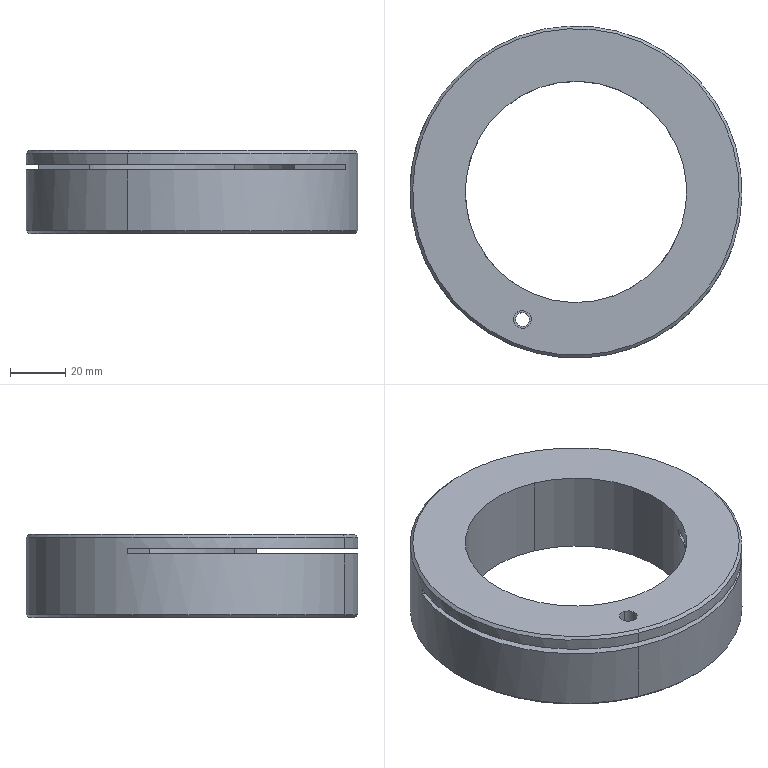Component | SolidWorks | 8TC-A17001-20-07LockingSleeve-1 | 1 solid | 34 faces | box 120 x 120 x 30 mm | volume 180598 mm3 | cylinder 16 | cone 12 | plane 6 | commonest cylinder face diameters 3.3 x8 5 x2 6.4 x2 80 x2 120 x2 | material #45
build123d program:
from build123d import *

# Parameters (mm, degrees)
SKETCH1_R                      = 60
SKETCH1_R_2                    = 40
BOSS_EXTRUDE1_DEPTH            = 15
SKETCH2_W                      = 60
SKETCH2_H                      = 2
CUT_EXTRUDE1_DEPTH             = 60
F_6_4_6_4_DIAMETER_HOLE1_D     = 6.4
F_6_4_6_4_DIAMETER_HOLE1_DEPTH = 5
M6_TAPPED_HOLE1_D              = 5
CHAMFER1_SIZE                  = 1
M4_TAPPED_HOLE1_D              = 3.3
M4_TAPPED_HOLE1_DEPTH          = 18
M4_TAPPED_HOLE1_TIP            = 0.9914


with BuildPart() as part:
    # Sketch1 → Boss-Extrude1 (new, symmetric)
    with BuildSketch(Plane(origin=(0, 0, 0), x_dir=(1, 0, 0), z_dir=(0, 1, 0))):
        with Locations(Location((0, 0, 0), (0, 0, 270))):
            Circle(SKETCH1_R)
        with Locations(Location((0, 0, 0), (0, 0, 270))):
            Circle(SKETCH1_R_2, mode=Mode.SUBTRACT)
    extrude(amount=BOSS_EXTRUDE1_DEPTH, both=True)

    # Sketch2 → Cut-Extrude1 (cut, symmetric)
    with BuildSketch(Plane(origin=(0, 0, 0), x_dir=(0, 0, -1), z_dir=(1, 0, 0))):
        with Locations((-30, 9)):
            Rectangle(SKETCH2_W, SKETCH2_H)
    extrude(amount=CUT_EXTRUDE1_DEPTH, both=True, mode=Mode.SUBTRACT)

    # 6.4 _6.4_ Diameter Hole1
    with Locations(Plane(origin=(0, 15, 0), x_dir=(1, 0, 0), z_dir=(0, 1, 0))):
        with Locations((0, -50)):
            Hole(F_6_4_6_4_DIAMETER_HOLE1_D / 2, depth=F_6_4_6_4_DIAMETER_HOLE1_DEPTH)

    # M6 Tapped Hole1 (through all)
    with Locations(Plane(origin=(0, 8, 0), x_dir=(1, 0, 0), z_dir=(0, 1, 0))):
        with Locations((0, -50)):
            Hole(M6_TAPPED_HOLE1_D / 2)

    # Chamfer1
    chamfer1_edges = [part.edges().sort_by_distance(p)[0] for p in [
        (0, -15, -60),
        (0, 15, -60),
    ]]
    chamfer(chamfer1_edges, length=CHAMFER1_SIZE)

    # M4 Tapped Hole1
    with Locations(Plane(origin=(0, -15, 0), x_dir=(-1, 0, 0), z_dir=(0, -1, 0))):
        with Locations((-35.355, 35.355), (35.355, 35.355), (35.355, -35.355), (-35.355, -35.355)):
            Hole(M4_TAPPED_HOLE1_D / 2, depth=M4_TAPPED_HOLE1_DEPTH)
            with Locations((0, 0, -(M4_TAPPED_HOLE1_DEPTH + M4_TAPPED_HOLE1_TIP / 2))):  # 118° drill point
                Cone(0, M4_TAPPED_HOLE1_D / 2, M4_TAPPED_HOLE1_TIP, mode=Mode.SUBTRACT)


solid = part.part

# Placed as in the assembly
solid = solid.moved(Location((733.029, 200.722, 253.5), (90, -22.788, 0)))
STEP:
#1=COLOUR_RGB('',0.7922,0.8196,0.9333);
#2=FILL_AREA_STYLE_COLOUR('',#1);
#3=FILL_AREA_STYLE('',(#2));
#4=SURFACE_STYLE_FILL_AREA(#3);
#5=SURFACE_SIDE_STYLE('',(#4));
#6=SURFACE_STYLE_USAGE(.BOTH.,#5);
#7=PRESENTATION_STYLE_ASSIGNMENT((#6));
#8=CARTESIAN_POINT('',(30.657,8.587,10.098));
#9=VERTEX_POINT('',#8);
#10=CARTESIAN_POINT('',(30.707,8.706,10.098));
#11=VERTEX_POINT('',#10);
#12=CARTESIAN_POINT('',(30.682,8.647,10.098));
#13=DIRECTION('',(-0.,-0.,-1.));
#14=DIRECTION('',(0.3873,0.9219,0.));
#15=AXIS2_PLACEMENT_3D('',#12,#13,#14);
#16=CIRCLE('',#15,0.06496);
#17=EDGE_CURVE('',#9,#11,#16,.T.);
#18=ORIENTED_EDGE('',*,*,#17,.F.);
#19=CARTESIAN_POINT('',(30.657,8.587,9.39));
#20=VERTEX_POINT('',#19);
#21=CARTESIAN_POINT('',(30.657,8.587,9.39));
#22=DIRECTION('',(-0.,-0.,-1.));
#23=VECTOR('',#22,39.37);
#24=LINE('',#21,#23);
#25=EDGE_CURVE('',#9,#20,#24,.T.);
#26=ORIENTED_EDGE('',*,*,#25,.T.);
#27=CARTESIAN_POINT('',(30.707,8.706,9.39));
#28=VERTEX_POINT('',#27);
#29=CARTESIAN_POINT('',(30.682,8.647,9.39));
#30=DIRECTION('',(-0.,-0.,-1.));
#31=DIRECTION('',(0.3873,0.9219,0.));
#32=AXIS2_PLACEMENT_3D('',#29,#30,#31);
#33=CIRCLE('',#32,0.06496);
#34=EDGE_CURVE('',#20,#28,#33,.T.);
#35=ORIENTED_EDGE('',*,*,#34,.T.);
#36=CARTESIAN_POINT('',(30.707,8.706,9.39));
#37=DIRECTION('',(-0.,-0.,-1.));
#38=VECTOR('',#37,39.37);
#39=LINE('',#36,#38);
#40=EDGE_CURVE('',#11,#28,#39,.T.);
#41=ORIENTED_EDGE('',*,*,#40,.F.);
#42=EDGE_LOOP('',(#18,#26,#35,#41));
#43=FACE_OUTER_BOUND('',#42,.T.);
#44=CARTESIAN_POINT('',(30.682,8.647,9.39));
#45=DIRECTION('',(-0.,-0.,-1.));
#46=DIRECTION('',(0.3873,0.9219,0.));
#47=AXIS2_PLACEMENT_3D('',#44,#45,#46);
#48=CYLINDRICAL_SURFACE('',#47,0.06496);
#49=ADVANCED_FACE('',(#43),#48,.F.);
#50=CARTESIAN_POINT('',(30.682,8.647,10.137));
#51=VERTEX_POINT('',#50);
#52=CARTESIAN_POINT('',(30.707,8.706,10.098));
#53=DIRECTION('',(0.332,0.7903,-0.515));
#54=VECTOR('',#53,39.37);
#55=LINE('',#52,#54);
#56=EDGE_CURVE('',#51,#11,#55,.T.);
#57=ORIENTED_EDGE('',*,*,#56,.F.);
#58=CARTESIAN_POINT('',(30.657,8.587,10.098));
#59=DIRECTION('',(-0.332,-0.7903,-0.515));
#60=VECTOR('',#59,39.37);
#61=LINE('',#58,#60);
#62=EDGE_CURVE('',#51,#9,#61,.T.);
#63=ORIENTED_EDGE('',*,*,#62,.T.);
#64=ORIENTED_EDGE('',*,*,#17,.T.);
#65=EDGE_LOOP('',(#57,#63,#64));
#66=FACE_OUTER_BOUND('',#65,.T.);
#67=CARTESIAN_POINT('',(30.682,8.647,10.098));
#68=DIRECTION('',(-0.,-0.,-1.));
#69=DIRECTION('',(0.3873,0.9219,0.));
#70=AXIS2_PLACEMENT_3D('',#67,#68,#69);
#71=CONICAL_SURFACE('',#70,0.06496,1.03);
#72=ADVANCED_FACE('',(#66),#71,.F.);
#73=CARTESIAN_POINT('',(28.09,9.665,10.098));
#74=VERTEX_POINT('',#73);
#75=CARTESIAN_POINT('',(28.14,9.785,10.098));
#76=VERTEX_POINT('',#75);
#77=CARTESIAN_POINT('',(28.115,9.725,10.098));
#78=DIRECTION('',(-0.,-0.,-1.));
#79=DIRECTION('',(0.3873,0.9219,0.));
#80=AXIS2_PLACEMENT_3D('',#77,#78,#79);
#81=CIRCLE('',#80,0.06496);
#82=EDGE_CURVE('',#74,#76,#81,.T.);
#83=ORIENTED_EDGE('',*,*,#82,.F.);
#84=CARTESIAN_POINT('',(28.09,9.665,9.39));
#85=VERTEX_POINT('',#84);
#86=CARTESIAN_POINT('',(28.09,9.665,9.39));
#87=DIRECTION('',(-0.,-0.,-1.));
#88=VECTOR('',#87,39.37);
#89=LINE('',#86,#88);
#90=EDGE_CURVE('',#74,#85,#89,.T.);
#91=ORIENTED_EDGE('',*,*,#90,.T.);
#92=CARTESIAN_POINT('',(28.14,9.785,9.39));
#93=VERTEX_POINT('',#92);
#94=CARTESIAN_POINT('',(28.115,9.725,9.39));
#95=DIRECTION('',(-0.,-0.,-1.));
#96=DIRECTION('',(0.3873,0.9219,0.));
#97=AXIS2_PLACEMENT_3D('',#94,#95,#96);
#98=CIRCLE('',#97,0.06496);
#99=EDGE_CURVE('',#85,#93,#98,.T.);
#100=ORIENTED_EDGE('',*,*,#99,.T.);
#101=CARTESIAN_POINT('',(28.14,9.785,9.39));
#102=DIRECTION('',(-0.,-0.,-1.));
#103=VECTOR('',#102,39.37);
#104=LINE('',#101,#103);
#105=EDGE_CURVE('',#76,#93,#104,.T.);
#106=ORIENTED_EDGE('',*,*,#105,.F.);
#107=EDGE_LOOP('',(#83,#91,#100,#106));
#108=FACE_OUTER_BOUND('',#107,.T.);
#109=CARTESIAN_POINT('',(28.115,9.725,9.39));
#110=DIRECTION('',(-0.,-0.,-1.));
#111=DIRECTION('',(0.3873,0.9219,0.));
#112=AXIS2_PLACEMENT_3D('',#109,#110,#111);
#113=CYLINDRICAL_SURFACE('',#112,0.06496);
#114=ADVANCED_FACE('',(#108),#113,.F.);
#115=CARTESIAN_POINT('',(28.115,9.725,10.137));
#116=VERTEX_POINT('',#115);
#117=CARTESIAN_POINT('',(28.14,9.785,10.098));
#118=DIRECTION('',(0.332,0.7903,-0.515));
#119=VECTOR('',#118,39.37);
#120=LINE('',#117,#119);
#121=EDGE_CURVE('',#116,#76,#120,.T.);
#122=ORIENTED_EDGE('',*,*,#121,.F.);
#123=CARTESIAN_POINT('',(28.09,9.665,10.098));
#124=DIRECTION('',(-0.332,-0.7903,-0.515));
#125=VECTOR('',#124,39.37);
#126=LINE('',#123,#125);
#127=EDGE_CURVE('',#116,#74,#126,.T.);
#128=ORIENTED_EDGE('',*,*,#127,.T.);
#129=ORIENTED_EDGE('',*,*,#82,.T.);
#130=EDGE_LOOP('',(#122,#128,#129));
#131=FACE_OUTER_BOUND('',#130,.T.);
#132=CARTESIAN_POINT('',(28.115,9.725,10.098));
#133=DIRECTION('',(-0.,-0.,-1.));
#134=DIRECTION('',(0.3873,0.9219,0.));
#135=AXIS2_PLACEMENT_3D('',#132,#133,#134);
#136=CONICAL_SURFACE('',#135,0.06496,1.03);
#137=ADVANCED_FACE('',(#131),#136,.F.);
#138=CARTESIAN_POINT('',(27.012,7.098,10.098));
#139=VERTEX_POINT('',#138);
#140=CARTESIAN_POINT('',(27.062,7.218,10.098));
#141=VERTEX_POINT('',#140);
#142=CARTESIAN_POINT('',(27.037,7.158,10.098));
#143=DIRECTION('',(-0.,-0.,-1.));
#144=DIRECTION('',(0.3873,0.9219,0.));
#145=AXIS2_PLACEMENT_3D('',#142,#143,#144);
#146=CIRCLE('',#145,0.06496);
#147=EDGE_CURVE('',#139,#141,#146,.T.);
#148=ORIENTED_EDGE('',*,*,#147,.F.);
#149=CARTESIAN_POINT('',(27.012,7.098,9.39));
#150=VERTEX_POINT('',#149);
#151=CARTESIAN_POINT('',(27.012,7.098,9.39));
#152=DIRECTION('',(-0.,-0.,-1.));
#153=VECTOR('',#152,39.37);
#154=LINE('',#151,#153);
#155=EDGE_CURVE('',#139,#150,#154,.T.);
#156=ORIENTED_EDGE('',*,*,#155,.T.);
#157=CARTESIAN_POINT('',(27.062,7.218,9.39));
#158=VERTEX_POINT('',#157);
#159=CARTESIAN_POINT('',(27.037,7.158,9.39));
#160=DIRECTION('',(-0.,-0.,-1.));
#161=DIRECTION('',(0.3873,0.9219,0.));
#162=AXIS2_PLACEMENT_3D('',#159,#160,#161);
#163=CIRCLE('',#162,0.06496);
#164=EDGE_CURVE('',#150,#158,#163,.T.);
#165=ORIENTED_EDGE('',*,*,#164,.T.);
#166=CARTESIAN_POINT('',(27.062,7.218,9.39));
#167=DIRECTION('',(-0.,-0.,-1.));
#168=VECTOR('',#167,39.37);
#169=LINE('',#166,#168);
#170=EDGE_CURVE('',#141,#158,#169,.T.);
#171=ORIENTED_EDGE('',*,*,#170,.F.);
#172=EDGE_LOOP('',(#148,#156,#165,#171));
#173=FACE_OUTER_BOUND('',#172,.T.);
#174=CARTESIAN_POINT('',(27.037,7.158,9.39));
#175=DIRECTION('',(-0.,-0.,-1.));
#176=DIRECTION('',(0.3873,0.9219,0.));
#177=AXIS2_PLACEMENT_3D('',#174,#175,#176);
#178=CYLINDRICAL_SURFACE('',#177,0.06496);
#179=ADVANCED_FACE('',(#173),#178,.F.);
#180=CARTESIAN_POINT('',(27.037,7.158,10.137));
#181=VERTEX_POINT('',#180);
#182=CARTESIAN_POINT('',(27.062,7.218,10.098));
#183=DIRECTION('',(0.332,0.7903,-0.515));
#184=VECTOR('',#183,39.37);
#185=LINE('',#182,#184);
#186=EDGE_CURVE('',#181,#141,#185,.T.);
#187=ORIENTED_EDGE('',*,*,#186,.F.);
#188=CARTESIAN_POINT('',(27.012,7.098,10.098));
#189=DIRECTION('',(-0.332,-0.7903,-0.515));
#190=VECTOR('',#189,39.37);
#191=LINE('',#188,#190);
#192=EDGE_CURVE('',#181,#139,#191,.T.);
#193=ORIENTED_EDGE('',*,*,#192,.T.);
#194=ORIENTED_EDGE('',*,*,#147,.T.);
#195=EDGE_LOOP('',(#187,#193,#194));
#196=FACE_OUTER_BOUND('',#195,.T.);
#197=CARTESIAN_POINT('',(27.037,7.158,10.098));
#198=DIRECTION('',(-0.,-0.,-1.));
#199=DIRECTION('',(0.3873,0.9219,0.));
#200=AXIS2_PLACEMENT_3D('',#197,#198,#199);
#201=CONICAL_SURFACE('',#200,0.06496,1.03);
#202=ADVANCED_FACE('',(#196),#201,.F.);
#203=CARTESIAN_POINT('',(29.578,6.02,10.098));
#204=VERTEX_POINT('',#203);
#205=CARTESIAN_POINT('',(29.629,6.14,10.098));
#206=VERTEX_POINT('',#205);
#207=CARTESIAN_POINT('',(29.604,6.08,10.098));
#208=DIRECTION('',(-0.,-0.,-1.));
#209=DIRECTION('',(0.3873,0.9219,0.));
#210=AXIS2_PLACEMENT_3D('',#207,#208,#209);
#211=CIRCLE('',#210,0.06496);
#212=EDGE_CURVE('',#204,#206,#211,.T.);
#213=ORIENTED_EDGE('',*,*,#212,.F.);
#214=CARTESIAN_POINT('',(29.578,6.02,9.39));
#215=VERTEX_POINT('',#214);
#216=CARTESIAN_POINT('',(29.578,6.02,9.39));
#217=DIRECTION('',(-0.,-0.,-1.));
#218=VECTOR('',#217,39.37);
#219=LINE('',#216,#218);
#220=EDGE_CURVE('',#204,#215,#219,.T.);
#221=ORIENTED_EDGE('',*,*,#220,.T.);
#222=CARTESIAN_POINT('',(29.629,6.14,9.39));
#223=VERTEX_POINT('',#222);
#224=CARTESIAN_POINT('',(29.604,6.08,9.39));
#225=DIRECTION('',(-0.,-0.,-1.));
#226=DIRECTION('',(0.3873,0.9219,0.));
#227=AXIS2_PLACEMENT_3D('',#224,#225,#226);
#228=CIRCLE('',#227,0.06496);
#229=EDGE_CURVE('',#215,#223,#228,.T.);
#230=ORIENTED_EDGE('',*,*,#229,.T.);
#231=CARTESIAN_POINT('',(29.629,6.14,9.39));
#232=DIRECTION('',(-0.,-0.,-1.));
#233=VECTOR('',#232,39.37);
#234=LINE('',#231,#233);
#235=EDGE_CURVE('',#206,#223,#234,.T.);
#236=ORIENTED_EDGE('',*,*,#235,.F.);
#237=EDGE_LOOP('',(#213,#221,#230,#236));
#238=FACE_OUTER_BOUND('',#237,.T.);
#239=CARTESIAN_POINT('',(29.604,6.08,9.39));
#240=DIRECTION('',(-0.,-0.,-1.));
#241=DIRECTION('',(0.3873,0.9219,0.));
#242=AXIS2_PLACEMENT_3D('',#239,#240,#241);
#243=CYLINDRICAL_SURFACE('',#242,0.06496);
#244=ADVANCED_FACE('',(#238),#243,.F.);
#245=CARTESIAN_POINT('',(29.604,6.08,10.137));
#246=VERTEX_POINT('',#245);
#247=CARTESIAN_POINT('',(29.629,6.14,10.098));
#248=DIRECTION('',(0.332,0.7903,-0.515));
#249=VECTOR('',#248,39.37);
#250=LINE('',#247,#249);
#251=EDGE_CURVE('',#246,#206,#250,.T.);
#252=ORIENTED_EDGE('',*,*,#251,.F.);
#253=CARTESIAN_POINT('',(29.578,6.02,10.098));
#254=DIRECTION('',(-0.332,-0.7903,-0.515));
#255=VECTOR('',#254,39.37);
#256=LINE('',#253,#255);
#257=EDGE_CURVE('',#246,#204,#256,.T.);
#258=ORIENTED_EDGE('',*,*,#257,.T.);
#259=ORIENTED_EDGE('',*,*,#212,.T.);
#260=EDGE_LOOP('',(#252,#258,#259));
#261=FACE_OUTER_BOUND('',#260,.T.);
#262=CARTESIAN_POINT('',(29.604,6.08,10.098));
#263=DIRECTION('',(-0.,-0.,-1.));
#264=DIRECTION('',(0.3873,0.9219,0.));
#265=AXIS2_PLACEMENT_3D('',#262,#263,#264);
#266=CONICAL_SURFACE('',#265,0.06496,1.03);
#267=ADVANCED_FACE('',(#261),#266,.F.);
#268=CARTESIAN_POINT('',(27.96,5.761,10.571));
#269=VERTEX_POINT('',#268);
#270=CARTESIAN_POINT('',(29.759,10.044,10.571));
#271=VERTEX_POINT('',#270);
#272=CARTESIAN_POINT('',(28.859,7.902,10.571));
#273=DIRECTION('',(0.,0.,1.));
#274=DIRECTION('',(-0.3873,-0.9219,0.));
#275=AXIS2_PLACEMENT_3D('',#272,#273,#274);
#276=CIRCLE('',#275,2.323);
#277=EDGE_CURVE('',#269,#271,#276,.T.);
#278=ORIENTED_EDGE('',*,*,#277,.F.);
#279=CARTESIAN_POINT('',(27.944,5.725,10.531));
#280=VERTEX_POINT('',#279);
#281=CARTESIAN_POINT('',(27.96,5.761,10.571));
#282=DIRECTION('',(-0.2739,-0.6519,-0.7071));
#283=VECTOR('',#282,39.37);
#284=LINE('',#281,#283);
#285=EDGE_CURVE('',#269,#280,#284,.T.);
#286=ORIENTED_EDGE('',*,*,#285,.T.);
#287=CARTESIAN_POINT('',(29.774,10.08,10.531));
#288=VERTEX_POINT('',#287);
#289=CARTESIAN_POINT('',(28.859,7.902,10.531));
#290=DIRECTION('',(-0.,-0.,-1.));
#291=DIRECTION('',(-0.3873,-0.9219,0.));
#292=AXIS2_PLACEMENT_3D('',#289,#290,#291);
#293=CIRCLE('',#292,2.362);
#294=EDGE_CURVE('',#288,#280,#293,.T.);
#295=ORIENTED_EDGE('',*,*,#294,.F.);
#296=CARTESIAN_POINT('',(29.759,10.044,10.571));
#297=DIRECTION('',(0.2739,0.6519,-0.7071));
#298=VECTOR('',#297,39.37);
#299=LINE('',#296,#298);
#300=EDGE_CURVE('',#271,#288,#299,.T.);
#301=ORIENTED_EDGE('',*,*,#300,.F.);
#302=EDGE_LOOP('',(#278,#286,#295,#301));
#303=FACE_OUTER_BOUND('',#302,.T.);
#304=CARTESIAN_POINT('',(28.859,7.902,10.571));
#305=DIRECTION('',(-0.,-0.,-1.));
#306=DIRECTION('',(0.3873,0.9219,0.));
#307=AXIS2_PLACEMENT_3D('',#304,#305,#306);
#308=CONICAL_SURFACE('',#307,2.323,0.7854);
#309=ADVANCED_FACE('',(#303),#308,.T.);
#310=CARTESIAN_POINT('',(29.759,10.044,9.39));
#311=VERTEX_POINT('',#310);
#312=CARTESIAN_POINT('',(27.96,5.761,9.39));
#313=VERTEX_POINT('',#312);
#314=CARTESIAN_POINT('',(28.859,7.902,9.39));
#315=DIRECTION('',(-0.,-0.,-1.));
#316=DIRECTION('',(-0.3873,-0.9219,0.));
#317=AXIS2_PLACEMENT_3D('',#314,#315,#316);
#318=CIRCLE('',#317,2.323);
#319=EDGE_CURVE('',#311,#313,#318,.T.);
#320=ORIENTED_EDGE('',*,*,#319,.F.);
#321=CARTESIAN_POINT('',(29.774,10.08,9.429));
#322=VERTEX_POINT('',#321);
#323=CARTESIAN_POINT('',(29.774,10.08,9.429));
#324=DIRECTION('',(0.2739,0.6519,0.7071));
#325=VECTOR('',#324,39.37);
#326=LINE('',#323,#325);
#327=EDGE_CURVE('',#311,#322,#326,.T.);
#328=ORIENTED_EDGE('',*,*,#327,.T.);
#329=CARTESIAN_POINT('',(27.944,5.725,9.429));
#330=VERTEX_POINT('',#329);
#331=CARTESIAN_POINT('',(28.859,7.902,9.429));
#332=DIRECTION('',(0.,0.,1.));
#333=DIRECTION('',(-0.3873,-0.9219,0.));
#334=AXIS2_PLACEMENT_3D('',#331,#332,#333);
#335=CIRCLE('',#334,2.362);
#336=EDGE_CURVE('',#330,#322,#335,.T.);
#337=ORIENTED_EDGE('',*,*,#336,.F.);
#338=CARTESIAN_POINT('',(27.944,5.725,9.429));
#339=DIRECTION('',(-0.2739,-0.6519,0.7071));
#340=VECTOR('',#339,39.37);
#341=LINE('',#338,#340);
#342=EDGE_CURVE('',#313,#330,#341,.T.);
#343=ORIENTED_EDGE('',*,*,#342,.F.);
#344=EDGE_LOOP('',(#320,#328,#337,#343));
#345=FACE_OUTER_BOUND('',#344,.T.);
#346=CARTESIAN_POINT('',(28.859,7.902,9.429));
#347=DIRECTION('',(0.,0.,1.));
#348=DIRECTION('',(-0.3873,-0.9219,0.));
#349=AXIS2_PLACEMENT_3D('',#346,#347,#348);
#350=CONICAL_SURFACE('',#349,2.362,0.7854);
#351=ADVANCED_FACE('',(#345),#350,.T.);
#352=CARTESIAN_POINT('',(28.135,6.178,9.39));
#353=VERTEX_POINT('',#352);
#354=CARTESIAN_POINT('',(28.059,5.997,9.39));
#355=VERTEX_POINT('',#354);
#356=CARTESIAN_POINT('',(28.097,6.088,9.39));
#357=DIRECTION('',(0.,0.,1.));
#358=DIRECTION('',(-0.3873,-0.9219,0.));
#359=AXIS2_PLACEMENT_3D('',#356,#357,#358);
#360=CIRCLE('',#359,0.09843);
#361=EDGE_CURVE('',#353,#355,#360,.T.);
#362=ORIENTED_EDGE('',*,*,#361,.F.);
#363=CARTESIAN_POINT('',(28.135,6.178,10.295));
#364=VERTEX_POINT('',#363);
#365=CARTESIAN_POINT('',(28.135,6.178,10.295));
#366=DIRECTION('',(0.,0.,1.));
#367=VECTOR('',#366,39.37);
#368=LINE('',#365,#367);
#369=EDGE_CURVE('',#353,#364,#368,.T.);
#370=ORIENTED_EDGE('',*,*,#369,.T.);
#371=CARTESIAN_POINT('',(28.059,5.997,10.295));
#372=VERTEX_POINT('',#371);
#373=CARTESIAN_POINT('',(28.097,6.088,10.295));
#374=DIRECTION('',(0.,0.,1.));
#375=DIRECTION('',(-0.3873,-0.9219,0.));
#376=AXIS2_PLACEMENT_3D('',#373,#374,#375);
#377=CIRCLE('',#376,0.09843);
#378=EDGE_CURVE('',#364,#372,#377,.T.);
#379=ORIENTED_EDGE('',*,*,#378,.T.);
#380=CARTESIAN_POINT('',(28.059,5.997,10.295));
#381=DIRECTION('',(0.,0.,1.));
#382=VECTOR('',#381,39.37);
#383=LINE('',#380,#382);
#384=EDGE_CURVE('',#355,#372,#383,.T.);
#385=ORIENTED_EDGE('',*,*,#384,.F.);
#386=EDGE_LOOP('',(#362,#370,#379,#385));
#387=FACE_OUTER_BOUND('',#386,.T.);
#388=CARTESIAN_POINT('',(28.097,6.088,10.295));
#389=DIRECTION('',(0.,0.,1.));
#390=DIRECTION('',(-0.3873,-0.9219,0.));
#391=AXIS2_PLACEMENT_3D('',#388,#389,#390);
#392=CYLINDRICAL_SURFACE('',#391,0.09843);
#393=ADVANCED_FACE('',(#387),#392,.F.);
#394=CARTESIAN_POINT('',(28.146,6.204,10.374));
#395=VERTEX_POINT('',#394);
#396=CARTESIAN_POINT('',(28.048,5.971,10.374));
#397=VERTEX_POINT('',#396);
#398=CARTESIAN_POINT('',(28.097,6.088,10.374));
#399=DIRECTION('',(0.,0.,1.));
#400=DIRECTION('',(-0.3873,-0.9219,0.));
#401=AXIS2_PLACEMENT_3D('',#398,#399,#400);
#402=CIRCLE('',#401,0.126);
#403=EDGE_CURVE('',#395,#397,#402,.T.);
#404=ORIENTED_EDGE('',*,*,#403,.F.);
#405=CARTESIAN_POINT('',(28.146,6.204,10.571));
#406=VERTEX_POINT('',#405);
#407=CARTESIAN_POINT('',(28.146,6.204,10.571));
#408=DIRECTION('',(0.,0.,1.));
#409=VECTOR('',#408,39.37);
#410=LINE('',#407,#409);
#411=EDGE_CURVE('',#395,#406,#410,.T.);
#412=ORIENTED_EDGE('',*,*,#411,.T.);
#413=CARTESIAN_POINT('',(28.048,5.971,10.571));
#414=VERTEX_POINT('',#413);
#415=CARTESIAN_POINT('',(28.097,6.088,10.571));
#416=DIRECTION('',(0.,0.,1.));
#417=DIRECTION('',(-0.3873,-0.9219,0.));
#418=AXIS2_PLACEMENT_3D('',#415,#416,#417);
#419=CIRCLE('',#418,0.126);
#420=EDGE_CURVE('',#406,#414,#419,.T.);
#421=ORIENTED_EDGE('',*,*,#420,.T.);
#422=CARTESIAN_POINT('',(28.048,5.971,10.571));
#423=DIRECTION('',(0.,0.,1.));
#424=VECTOR('',#423,39.37);
#425=LINE('',#422,#424);
#426=EDGE_CURVE('',#397,#414,#425,.T.);
#427=ORIENTED_EDGE('',*,*,#426,.F.);
#428=EDGE_LOOP('',(#404,#412,#421,#427));
#429=FACE_OUTER_BOUND('',#428,.T.);
#430=CARTESIAN_POINT('',(28.097,6.088,10.571));
#431=DIRECTION('',(0.,0.,1.));
#432=DIRECTION('',(-0.3873,-0.9219,0.));
#433=AXIS2_PLACEMENT_3D('',#430,#431,#432);
#434=CYLINDRICAL_SURFACE('',#433,0.126);
#435=ADVANCED_FACE('',(#429),#434,.F.);
#436=CARTESIAN_POINT('',(29.469,9.354,10.571));
#437=VERTEX_POINT('',#436);
#438=CARTESIAN_POINT('',(28.249,6.451,10.571));
#439=VERTEX_POINT('',#438);
#440=CARTESIAN_POINT('',(28.859,7.902,10.571));
#441=DIRECTION('',(0.,0.,1.));
#442=DIRECTION('',(-0.3873,-0.9219,0.));
#443=AXIS2_PLACEMENT_3D('',#440,#441,#442);
#444=CIRCLE('',#443,1.575);
#445=EDGE_CURVE('',#437,#439,#444,.T.);
#446=ORIENTED_EDGE('',*,*,#445,.T.);
#447=CARTESIAN_POINT('',(28.249,6.451,10.374));
#448=VERTEX_POINT('',#447);
#449=CARTESIAN_POINT('',(28.249,6.451,10.571));
#450=DIRECTION('',(-0.,-0.,-1.));
#451=VECTOR('',#450,39.37);
#452=LINE('',#449,#451);
#453=EDGE_CURVE('',#439,#448,#452,.T.);
#454=ORIENTED_EDGE('',*,*,#453,.T.);
#455=CARTESIAN_POINT('',(27.408,8.512,10.374));
#456=VERTEX_POINT('',#455);
#457=CARTESIAN_POINT('',(28.859,7.902,10.374));
#458=DIRECTION('',(0.,0.,1.));
#459=DIRECTION('',(-0.3873,-0.9219,0.));
#460=AXIS2_PLACEMENT_3D('',#457,#458,#459);
#461=CIRCLE('',#460,1.575);
#462=EDGE_CURVE('',#456,#448,#461,.T.);
#463=ORIENTED_EDGE('',*,*,#462,.F.);
#464=CARTESIAN_POINT('',(27.408,8.512,10.295));
#465=VERTEX_POINT('',#464);
#466=CARTESIAN_POINT('',(27.408,8.512,10.571));
#467=DIRECTION('',(0.,0.,1.));
#468=VECTOR('',#467,39.37);
#469=LINE('',#466,#468);
#470=EDGE_CURVE('',#465,#456,#469,.T.);
#471=ORIENTED_EDGE('',*,*,#470,.F.);
#472=CARTESIAN_POINT('',(28.249,6.451,10.295));
#473=VERTEX_POINT('',#472);
#474=CARTESIAN_POINT('',(28.859,7.902,10.295));
#475=DIRECTION('',(-0.,-0.,-1.));
#476=DIRECTION('',(0.3873,0.9219,0.));
#477=AXIS2_PLACEMENT_3D('',#474,#475,#476);
#478=CIRCLE('',#477,1.575);
#479=EDGE_CURVE('',#473,#465,#478,.T.);
#480=ORIENTED_EDGE('',*,*,#479,.F.);
#481=CARTESIAN_POINT('',(28.249,6.451,9.39));
#482=VERTEX_POINT('',#481);
#483=CARTESIAN_POINT('',(28.249,6.451,10.571));
#484=DIRECTION('',(-0.,-0.,-1.));
#485=VECTOR('',#484,39.37);
#486=LINE('',#483,#485);
#487=EDGE_CURVE('',#473,#482,#486,.T.);
#488=ORIENTED_EDGE('',*,*,#487,.T.);
#489=CARTESIAN_POINT('',(29.469,9.354,9.39));
#490=VERTEX_POINT('',#489);
#491=CARTESIAN_POINT('',(28.859,7.902,9.39));
#492=DIRECTION('',(0.,0.,1.));
#493=DIRECTION('',(-0.3873,-0.9219,0.));
#494=AXIS2_PLACEMENT_3D('',#491,#492,#493);
#495=CIRCLE('',#494,1.575);
#496=EDGE_CURVE('',#490,#482,#495,.T.);
#497=ORIENTED_EDGE('',*,*,#496,.F.);
#498=CARTESIAN_POINT('',(29.469,9.354,10.571));
#499=DIRECTION('',(-0.,-0.,-1.));
#500=VECTOR('',#499,39.37);
#501=LINE('',#498,#500);
#502=EDGE_CURVE('',#437,#490,#501,.T.);
#503=ORIENTED_EDGE('',*,*,#502,.F.);
#504=EDGE_LOOP('',(#446,#454,#463,#471,#480,#488,#497,#503));
#505=FACE_OUTER_BOUND('',#504,.T.);
#506=CARTESIAN_POINT('',(28.859,7.902,10.571));
#507=DIRECTION('',(-0.,-0.,-1.));
#508=DIRECTION('',(0.3873,0.9219,0.));
#509=AXIS2_PLACEMENT_3D('',#506,#507,#508);
#510=CYLINDRICAL_SURFACE('',#509,1.575);
#511=ADVANCED_FACE('',(#505),#510,.F.);
#512=ORIENTED_EDGE('',*,*,#294,.T.);
#513=CARTESIAN_POINT('',(27.944,5.725,10.374));
#514=VERTEX_POINT('',#513);
#515=CARTESIAN_POINT('',(27.944,5.725,10.571));
#516=DIRECTION('',(-0.,-0.,-1.));
#517=VECTOR('',#516,39.37);
#518=LINE('',#515,#517);
#519=EDGE_CURVE('',#280,#514,#518,.T.);
#520=ORIENTED_EDGE('',*,*,#519,.T.);
#521=CARTESIAN_POINT('',(31.037,6.987,10.374));
#522=VERTEX_POINT('',#521);
#523=CARTESIAN_POINT('',(28.859,7.902,10.374));
#524=DIRECTION('',(0.,0.,1.));
#525=DIRECTION('',(-0.3873,-0.9219,0.));
#526=AXIS2_PLACEMENT_3D('',#523,#524,#525);
#527=CIRCLE('',#526,2.362);
#528=EDGE_CURVE('',#514,#522,#527,.T.);
#529=ORIENTED_EDGE('',*,*,#528,.T.);
#530=CARTESIAN_POINT('',(31.037,6.987,10.295));
#531=VERTEX_POINT('',#530);
#532=CARTESIAN_POINT('',(31.037,6.987,10.374));
#533=DIRECTION('',(0.,0.,1.));
#534=VECTOR('',#533,39.37);
#535=LINE('',#532,#534);
#536=EDGE_CURVE('',#531,#522,#535,.T.);
#537=ORIENTED_EDGE('',*,*,#536,.F.);
#538=CARTESIAN_POINT('',(27.944,5.725,10.295));
#539=VERTEX_POINT('',#538);
#540=CARTESIAN_POINT('',(28.859,7.902,10.295));
#541=DIRECTION('',(-0.,-0.,-1.));
#542=DIRECTION('',(0.3873,0.9219,0.));
#543=AXIS2_PLACEMENT_3D('',#540,#541,#542);
#544=CIRCLE('',#543,2.362);
#545=EDGE_CURVE('',#531,#539,#544,.T.);
#546=ORIENTED_EDGE('',*,*,#545,.T.);
#547=CARTESIAN_POINT('',(27.944,5.725,10.571));
#548=DIRECTION('',(-0.,-0.,-1.));
#549=VECTOR('',#548,39.37);
#550=LINE('',#547,#549);
#551=EDGE_CURVE('',#539,#330,#550,.T.);
#552=ORIENTED_EDGE('',*,*,#551,.T.);
#553=ORIENTED_EDGE('',*,*,#336,.T.);
#554=CARTESIAN_POINT('',(29.774,10.08,10.571));
#555=DIRECTION('',(-0.,-0.,-1.));
#556=VECTOR('',#555,39.37);
#557=LINE('',#554,#556);
#558=EDGE_CURVE('',#288,#322,#557,.T.);
#559=ORIENTED_EDGE('',*,*,#558,.F.);
#560=EDGE_LOOP('',(#512,#520,#529,#537,#546,#552,#553,#559));
#561=FACE_OUTER_BOUND('',#560,.T.);
#562=CARTESIAN_POINT('',(28.859,7.902,10.571));
#563=DIRECTION('',(-0.,-0.,-1.));
#564=DIRECTION('',(0.3873,0.9219,0.));
#565=AXIS2_PLACEMENT_3D('',#562,#563,#564);
#566=CYLINDRICAL_SURFACE('',#565,2.362);
#567=ADVANCED_FACE('',(#561),#566,.T.);
#568=CARTESIAN_POINT('',(28.859,7.902,10.571));
#569=DIRECTION('',(0.,0.,1.));
#570=DIRECTION('',(-0.3873,-0.9219,0.));
#571=AXIS2_PLACEMENT_3D('',#568,#569,#570);
#572=CIRCLE('',#571,2.323);
#573=EDGE_CURVE('',#271,#269,#572,.T.);
#574=ORIENTED_EDGE('',*,*,#573,.T.);
#575=ORIENTED_EDGE('',*,*,#277,.T.);
#576=EDGE_LOOP('',(#574,#575));
#577=FACE_OUTER_BOUND('',#576,.T.);
#578=CARTESIAN_POINT('',(28.097,6.088,10.571));
#579=DIRECTION('',(0.,0.,1.));
#580=DIRECTION('',(-0.3873,-0.9219,0.));
#581=AXIS2_PLACEMENT_3D('',#578,#579,#580);
#582=CIRCLE('',#581,0.126);
#583=EDGE_CURVE('',#414,#406,#582,.T.);
#584=ORIENTED_EDGE('',*,*,#583,.F.);
#585=ORIENTED_EDGE('',*,*,#420,.F.);
#586=EDGE_LOOP('',(#584,#585));
#587=FACE_BOUND('',#586,.T.);
#588=ORIENTED_EDGE('',*,*,#445,.F.);
#589=CARTESIAN_POINT('',(28.859,7.902,10.571));
#590=DIRECTION('',(0.,0.,1.));
#591=DIRECTION('',(-0.3873,-0.9219,0.));
#592=AXIS2_PLACEMENT_3D('',#589,#590,#591);
#593=CIRCLE('',#592,1.575);
#594=EDGE_CURVE('',#439,#437,#593,.T.);
#595=ORIENTED_EDGE('',*,*,#594,.F.);
#596=EDGE_LOOP('',(#588,#595));
#597=FACE_BOUND('',#596,.T.);
#598=CARTESIAN_POINT('',(28.859,7.902,10.571));
#599=DIRECTION('',(0.,0.,1.));
#600=DIRECTION('',(-0.3873,-0.9219,0.));
#601=AXIS2_PLACEMENT_3D('',#598,#599,#600);
#602=PLANE('',#601);
#603=ADVANCED_FACE('',(#577,#587,#597),#602,.T.);
#604=CARTESIAN_POINT('',(30.682,8.647,9.39));
#605=DIRECTION('',(-0.,-0.,-1.));
#606=DIRECTION('',(0.3873,0.9219,0.));
#607=AXIS2_PLACEMENT_3D('',#604,#605,#606);
#608=CIRCLE('',#607,0.06496);
#609=EDGE_CURVE('',#28,#20,#608,.T.);
#610=ORIENTED_EDGE('',*,*,#609,.F.);
#611=ORIENTED_EDGE('',*,*,#34,.F.);
#612=EDGE_LOOP('',(#610,#611));
#613=FACE_BOUND('',#612,.T.);
#614=CARTESIAN_POINT('',(28.115,9.725,9.39));
#615=DIRECTION('',(-0.,-0.,-1.));
#616=DIRECTION('',(0.3873,0.9219,0.));
#617=AXIS2_PLACEMENT_3D('',#614,#615,#616);
#618=CIRCLE('',#617,0.06496);
#619=EDGE_CURVE('',#93,#85,#618,.T.);
#620=ORIENTED_EDGE('',*,*,#619,.F.);
#621=ORIENTED_EDGE('',*,*,#99,.F.);
#622=EDGE_LOOP('',(#620,#621));
#623=FACE_BOUND('',#622,.T.);
#624=CARTESIAN_POINT('',(27.037,7.158,9.39));
#625=DIRECTION('',(-0.,-0.,-1.));
#626=DIRECTION('',(0.3873,0.9219,0.));
#627=AXIS2_PLACEMENT_3D('',#624,#625,#626);
#628=CIRCLE('',#627,0.06496);
#629=EDGE_CURVE('',#158,#150,#628,.T.);
#630=ORIENTED_EDGE('',*,*,#629,.F.);
#631=ORIENTED_EDGE('',*,*,#164,.F.);
#632=EDGE_LOOP('',(#630,#631));
#633=FACE_BOUND('',#632,.T.);
#634=CARTESIAN_POINT('',(29.604,6.08,9.39));
#635=DIRECTION('',(-0.,-0.,-1.));
#636=DIRECTION('',(0.3873,0.9219,0.));
#637=AXIS2_PLACEMENT_3D('',#634,#635,#636);
#638=CIRCLE('',#637,0.06496);
#639=EDGE_CURVE('',#223,#215,#638,.T.);
#640=ORIENTED_EDGE('',*,*,#639,.F.);
#641=ORIENTED_EDGE('',*,*,#229,.F.);
#642=EDGE_LOOP('',(#640,#641));
#643=FACE_BOUND('',#642,.T.);
#644=CARTESIAN_POINT('',(28.859,7.902,9.39));
#645=DIRECTION('',(-0.,-0.,-1.));
#646=DIRECTION('',(-0.3873,-0.9219,0.));
#647=AXIS2_PLACEMENT_3D('',#644,#645,#646);
#648=CIRCLE('',#647,2.323);
#649=EDGE_CURVE('',#313,#311,#648,.T.);
#650=ORIENTED_EDGE('',*,*,#649,.T.);
#651=ORIENTED_EDGE('',*,*,#319,.T.);
#652=EDGE_LOOP('',(#650,#651));
#653=FACE_OUTER_BOUND('',#652,.T.);
#654=CARTESIAN_POINT('',(28.097,6.088,9.39));
#655=DIRECTION('',(0.,0.,1.));
#656=DIRECTION('',(-0.3873,-0.9219,0.));
#657=AXIS2_PLACEMENT_3D('',#654,#655,#656);
#658=CIRCLE('',#657,0.09843);
#659=EDGE_CURVE('',#355,#353,#658,.T.);
#660=ORIENTED_EDGE('',*,*,#659,.T.);
#661=ORIENTED_EDGE('',*,*,#361,.T.);
#662=EDGE_LOOP('',(#660,#661));
#663=FACE_BOUND('',#662,.T.);
#664=ORIENTED_EDGE('',*,*,#496,.T.);
#665=CARTESIAN_POINT('',(28.859,7.902,9.39));
#666=DIRECTION('',(0.,0.,1.));
#667=DIRECTION('',(-0.3873,-0.9219,0.));
#668=AXIS2_PLACEMENT_3D('',#665,#666,#667);
#669=CIRCLE('',#668,1.575);
#670=EDGE_CURVE('',#482,#490,#669,.T.);
#671=ORIENTED_EDGE('',*,*,#670,.T.);
#672=EDGE_LOOP('',(#664,#671));
#673=FACE_BOUND('',#672,.T.);
#674=CARTESIAN_POINT('',(28.859,7.902,9.39));
#675=DIRECTION('',(0.,0.,1.));
#676=DIRECTION('',(-0.3873,-0.9219,0.));
#677=AXIS2_PLACEMENT_3D('',#674,#675,#676);
#678=PLANE('',#677);
#679=ADVANCED_FACE('',(#613,#623,#633,#643,#653,#663,#673),#678,.F.);
#680=ORIENTED_EDGE('',*,*,#519,.F.);
#681=CARTESIAN_POINT('',(28.859,7.902,10.531));
#682=DIRECTION('',(-0.,-0.,-1.));
#683=DIRECTION('',(-0.3873,-0.9219,0.));
#684=AXIS2_PLACEMENT_3D('',#681,#682,#683);
#685=CIRCLE('',#684,2.362);
#686=EDGE_CURVE('',#280,#288,#685,.T.);
#687=ORIENTED_EDGE('',*,*,#686,.T.);
#688=ORIENTED_EDGE('',*,*,#558,.T.);
#689=CARTESIAN_POINT('',(28.859,7.902,9.429));
#690=DIRECTION('',(0.,0.,1.));
#691=DIRECTION('',(-0.3873,-0.9219,0.));
#692=AXIS2_PLACEMENT_3D('',#689,#690,#691);
#693=CIRCLE('',#692,2.362);
#694=EDGE_CURVE('',#322,#330,#693,.T.);
#695=ORIENTED_EDGE('',*,*,#694,.T.);
#696=ORIENTED_EDGE('',*,*,#551,.F.);
#697=CARTESIAN_POINT('',(26.682,8.817,10.295));
#698=VERTEX_POINT('',#697);
#699=CARTESIAN_POINT('',(28.859,7.902,10.295));
#700=DIRECTION('',(-0.,-0.,-1.));
#701=DIRECTION('',(0.3873,0.9219,0.));
#702=AXIS2_PLACEMENT_3D('',#699,#700,#701);
#703=CIRCLE('',#702,2.362);
#704=EDGE_CURVE('',#539,#698,#703,.T.);
#705=ORIENTED_EDGE('',*,*,#704,.T.);
#706=CARTESIAN_POINT('',(26.682,8.817,10.374));
#707=VERTEX_POINT('',#706);
#708=CARTESIAN_POINT('',(26.682,8.817,10.374));
#709=DIRECTION('',(0.,0.,1.));
#710=VECTOR('',#709,39.37);
#711=LINE('',#708,#710);
#712=EDGE_CURVE('',#698,#707,#711,.T.);
#713=ORIENTED_EDGE('',*,*,#712,.T.);
#714=CARTESIAN_POINT('',(28.859,7.902,10.374));
#715=DIRECTION('',(0.,0.,1.));
#716=DIRECTION('',(-0.3873,-0.9219,0.));
#717=AXIS2_PLACEMENT_3D('',#714,#715,#716);
#718=CIRCLE('',#717,2.362);
#719=EDGE_CURVE('',#707,#514,#718,.T.);
#720=ORIENTED_EDGE('',*,*,#719,.T.);
#721=EDGE_LOOP('',(#680,#687,#688,#695,#696,#705,#713,#720));
#722=FACE_OUTER_BOUND('',#721,.T.);
#723=CARTESIAN_POINT('',(28.859,7.902,10.571));
#724=DIRECTION('',(-0.,-0.,-1.));
#725=DIRECTION('',(0.3873,0.9219,0.));
#726=AXIS2_PLACEMENT_3D('',#723,#724,#725);
#727=CYLINDRICAL_SURFACE('',#726,2.362);
#728=ADVANCED_FACE('',(#722),#727,.T.);
#729=ORIENTED_EDGE('',*,*,#453,.F.);
#730=ORIENTED_EDGE('',*,*,#594,.T.);
#731=ORIENTED_EDGE('',*,*,#502,.T.);
#732=ORIENTED_EDGE('',*,*,#670,.F.);
#733=ORIENTED_EDGE('',*,*,#487,.F.);
#734=CARTESIAN_POINT('',(30.311,7.292,10.295));
#735=VERTEX_POINT('',#734);
#736=CARTESIAN_POINT('',(28.859,7.902,10.295));
#737=DIRECTION('',(-0.,-0.,-1.));
#738=DIRECTION('',(0.3873,0.9219,0.));
#739=AXIS2_PLACEMENT_3D('',#736,#737,#738);
#740=CIRCLE('',#739,1.575);
#741=EDGE_CURVE('',#735,#473,#740,.T.);
#742=ORIENTED_EDGE('',*,*,#741,.F.);
#743=CARTESIAN_POINT('',(30.311,7.292,10.374));
#744=VERTEX_POINT('',#743);
#745=CARTESIAN_POINT('',(30.311,7.292,10.571));
#746=DIRECTION('',(-0.,-0.,-1.));
#747=VECTOR('',#746,39.37);
#748=LINE('',#745,#747);
#749=EDGE_CURVE('',#744,#735,#748,.T.);
#750=ORIENTED_EDGE('',*,*,#749,.F.);
#751=CARTESIAN_POINT('',(28.859,7.902,10.374));
#752=DIRECTION('',(0.,0.,1.));
#753=DIRECTION('',(-0.3873,-0.9219,0.));
#754=AXIS2_PLACEMENT_3D('',#751,#752,#753);
#755=CIRCLE('',#754,1.575);
#756=EDGE_CURVE('',#448,#744,#755,.T.);
#757=ORIENTED_EDGE('',*,*,#756,.F.);
#758=EDGE_LOOP('',(#729,#730,#731,#732,#733,#742,#750,#757));
#759=FACE_OUTER_BOUND('',#758,.T.);
#760=CARTESIAN_POINT('',(28.859,7.902,10.571));
#761=DIRECTION('',(-0.,-0.,-1.));
#762=DIRECTION('',(0.3873,0.9219,0.));
#763=AXIS2_PLACEMENT_3D('',#760,#761,#762);
#764=CYLINDRICAL_SURFACE('',#763,1.575);
#765=ADVANCED_FACE('',(#759),#764,.F.);
#766=CARTESIAN_POINT('',(28.097,6.088,10.374));
#767=DIRECTION('',(0.,0.,1.));
#768=DIRECTION('',(-0.3873,-0.9219,0.));
#769=AXIS2_PLACEMENT_3D('',#766,#767,#768);
#770=CIRCLE('',#769,0.126);
#771=EDGE_CURVE('',#397,#395,#770,.T.);
#772=ORIENTED_EDGE('',*,*,#771,.T.);
#773=ORIENTED_EDGE('',*,*,#403,.T.);
#774=EDGE_LOOP('',(#772,#773));
#775=FACE_BOUND('',#774,.T.);
#776=ORIENTED_EDGE('',*,*,#719,.F.);
#777=CARTESIAN_POINT('',(26.682,8.817,10.374));
#778=DIRECTION('',(0.9219,-0.3873,-0.));
#779=VECTOR('',#778,39.37);
#780=LINE('',#777,#779);
#781=EDGE_CURVE('',#707,#456,#780,.T.);
#782=ORIENTED_EDGE('',*,*,#781,.T.);
#783=ORIENTED_EDGE('',*,*,#462,.T.);
#784=ORIENTED_EDGE('',*,*,#756,.T.);
#785=CARTESIAN_POINT('',(26.682,8.817,10.374));
#786=DIRECTION('',(0.9219,-0.3873,-0.));
#787=VECTOR('',#786,39.37);
#788=LINE('',#785,#787);
#789=EDGE_CURVE('',#744,#522,#788,.T.);
#790=ORIENTED_EDGE('',*,*,#789,.T.);
#791=ORIENTED_EDGE('',*,*,#528,.F.);
#792=EDGE_LOOP('',(#776,#782,#783,#784,#790,#791));
#793=FACE_OUTER_BOUND('',#792,.T.);
#794=CARTESIAN_POINT('',(25.767,6.64,10.374));
#795=DIRECTION('',(0.,0.,1.));
#796=DIRECTION('',(-0.3873,-0.9219,0.));
#797=AXIS2_PLACEMENT_3D('',#794,#795,#796);
#798=PLANE('',#797);
#799=ADVANCED_FACE('',(#775,#793),#798,.F.);
#800=ORIENTED_EDGE('',*,*,#749,.T.);
#801=CARTESIAN_POINT('',(26.682,8.817,10.295));
#802=DIRECTION('',(0.9219,-0.3873,-0.));
#803=VECTOR('',#802,39.37);
#804=LINE('',#801,#803);
#805=EDGE_CURVE('',#735,#531,#804,.T.);
#806=ORIENTED_EDGE('',*,*,#805,.T.);
#807=ORIENTED_EDGE('',*,*,#536,.T.);
#808=ORIENTED_EDGE('',*,*,#789,.F.);
#809=EDGE_LOOP('',(#800,#806,#807,#808));
#810=FACE_OUTER_BOUND('',#809,.T.);
#811=CARTESIAN_POINT('',(26.682,8.817,10.374));
#812=DIRECTION('',(0.3873,0.9219,-0.));
#813=DIRECTION('',(-0.9219,0.3873,0.));
#814=AXIS2_PLACEMENT_3D('',#811,#812,#813);
#815=PLANE('',#814);
#816=ADVANCED_FACE('',(#810),#815,.F.);
#817=CARTESIAN_POINT('',(28.097,6.088,10.295));
#818=DIRECTION('',(0.,0.,1.));
#819=DIRECTION('',(-0.3873,-0.9219,0.));
#820=AXIS2_PLACEMENT_3D('',#817,#818,#819);
#821=CIRCLE('',#820,0.09843);
#822=EDGE_CURVE('',#372,#364,#821,.T.);
#823=ORIENTED_EDGE('',*,*,#822,.F.);
#824=ORIENTED_EDGE('',*,*,#378,.F.);
#825=EDGE_LOOP('',(#823,#824));
#826=FACE_BOUND('',#825,.T.);
#827=ORIENTED_EDGE('',*,*,#805,.F.);
#828=ORIENTED_EDGE('',*,*,#741,.T.);
#829=ORIENTED_EDGE('',*,*,#479,.T.);
#830=CARTESIAN_POINT('',(26.682,8.817,10.295));
#831=DIRECTION('',(0.9219,-0.3873,-0.));
#832=VECTOR('',#831,39.37);
#833=LINE('',#830,#832);
#834=EDGE_CURVE('',#698,#465,#833,.T.);
#835=ORIENTED_EDGE('',*,*,#834,.F.);
#836=ORIENTED_EDGE('',*,*,#704,.F.);
#837=ORIENTED_EDGE('',*,*,#545,.F.);
#838=EDGE_LOOP('',(#827,#828,#829,#835,#836,#837));
#839=FACE_OUTER_BOUND('',#838,.T.);
#840=CARTESIAN_POINT('',(25.767,6.64,10.295));
#841=DIRECTION('',(-0.,-0.,-1.));
#842=DIRECTION('',(0.3873,0.9219,-0.));
#843=AXIS2_PLACEMENT_3D('',#840,#841,#842);
#844=PLANE('',#843);
#845=ADVANCED_FACE('',(#826,#839),#844,.F.);
#846=ORIENTED_EDGE('',*,*,#470,.T.);
#847=ORIENTED_EDGE('',*,*,#781,.F.);
#848=ORIENTED_EDGE('',*,*,#712,.F.);
#849=ORIENTED_EDGE('',*,*,#834,.T.);
#850=EDGE_LOOP('',(#846,#847,#848,#849));
#851=FACE_OUTER_BOUND('',#850,.T.);
#852=CARTESIAN_POINT('',(26.682,8.817,10.374));
#853=DIRECTION('',(0.3873,0.9219,-0.));
#854=DIRECTION('',(-0.9219,0.3873,0.));
#855=AXIS2_PLACEMENT_3D('',#852,#853,#854);
#856=PLANE('',#855);
#857=ADVANCED_FACE('',(#851),#856,.F.);
#858=ORIENTED_EDGE('',*,*,#411,.F.);
#859=ORIENTED_EDGE('',*,*,#771,.F.);
#860=ORIENTED_EDGE('',*,*,#426,.T.);
#861=ORIENTED_EDGE('',*,*,#583,.T.);
#862=EDGE_LOOP('',(#858,#859,#860,#861));
#863=FACE_OUTER_BOUND('',#862,.T.);
#864=CARTESIAN_POINT('',(28.097,6.088,10.571));
#865=DIRECTION('',(0.,0.,1.));
#866=DIRECTION('',(-0.3873,-0.9219,0.));
#867=AXIS2_PLACEMENT_3D('',#864,#865,#866);
#868=CYLINDRICAL_SURFACE('',#867,0.126);
#869=ADVANCED_FACE('',(#863),#868,.F.);
#870=ORIENTED_EDGE('',*,*,#369,.F.);
#871=ORIENTED_EDGE('',*,*,#659,.F.);
#872=ORIENTED_EDGE('',*,*,#384,.T.);
#873=ORIENTED_EDGE('',*,*,#822,.T.);
#874=EDGE_LOOP('',(#870,#871,#872,#873));
#875=FACE_OUTER_BOUND('',#874,.T.);
#876=CARTESIAN_POINT('',(28.097,6.088,10.295));
#877=DIRECTION('',(0.,0.,1.));
#878=DIRECTION('',(-0.3873,-0.9219,0.));
#879=AXIS2_PLACEMENT_3D('',#876,#877,#878);
#880=CYLINDRICAL_SURFACE('',#879,0.09843);
#881=ADVANCED_FACE('',(#875),#880,.F.);
#882=ORIENTED_EDGE('',*,*,#327,.F.);
#883=ORIENTED_EDGE('',*,*,#649,.F.);
#884=ORIENTED_EDGE('',*,*,#342,.T.);
#885=ORIENTED_EDGE('',*,*,#694,.F.);
#886=EDGE_LOOP('',(#882,#883,#884,#885));
#887=FACE_OUTER_BOUND('',#886,.T.);
#888=CARTESIAN_POINT('',(28.859,7.902,9.429));
#889=DIRECTION('',(0.,0.,1.));
#890=DIRECTION('',(-0.3873,-0.9219,0.));
#891=AXIS2_PLACEMENT_3D('',#888,#889,#890);
#892=CONICAL_SURFACE('',#891,2.362,0.7854);
#893=ADVANCED_FACE('',(#887),#892,.T.);
#894=ORIENTED_EDGE('',*,*,#285,.F.);
#895=ORIENTED_EDGE('',*,*,#573,.F.);
#896=ORIENTED_EDGE('',*,*,#300,.T.);
#897=ORIENTED_EDGE('',*,*,#686,.F.);
#898=EDGE_LOOP('',(#894,#895,#896,#897));
#899=FACE_OUTER_BOUND('',#898,.T.);
#900=CARTESIAN_POINT('',(28.859,7.902,10.571));
#901=DIRECTION('',(-0.,-0.,-1.));
#902=DIRECTION('',(0.3873,0.9219,0.));
#903=AXIS2_PLACEMENT_3D('',#900,#901,#902);
#904=CONICAL_SURFACE('',#903,2.323,0.7854);
#905=ADVANCED_FACE('',(#899),#904,.T.);
#906=ORIENTED_EDGE('',*,*,#257,.F.);
#907=ORIENTED_EDGE('',*,*,#251,.T.);
#908=CARTESIAN_POINT('',(29.604,6.08,10.098));
#909=DIRECTION('',(-0.,-0.,-1.));
#910=DIRECTION('',(0.3873,0.9219,0.));
#911=AXIS2_PLACEMENT_3D('',#908,#909,#910);
#912=CIRCLE('',#911,0.06496);
#913=EDGE_CURVE('',#206,#204,#912,.T.);
#914=ORIENTED_EDGE('',*,*,#913,.T.);
#915=EDGE_LOOP('',(#906,#907,#914));
#916=FACE_OUTER_BOUND('',#915,.T.);
#917=CARTESIAN_POINT('',(29.604,6.08,10.098));
#918=DIRECTION('',(-0.,-0.,-1.));
#919=DIRECTION('',(0.3873,0.9219,0.));
#920=AXIS2_PLACEMENT_3D('',#917,#918,#919);
#921=CONICAL_SURFACE('',#920,0.06496,1.03);
#922=ADVANCED_FACE('',(#916),#921,.F.);
#923=ORIENTED_EDGE('',*,*,#220,.F.);
#924=ORIENTED_EDGE('',*,*,#913,.F.);
#925=ORIENTED_EDGE('',*,*,#235,.T.);
#926=ORIENTED_EDGE('',*,*,#639,.T.);
#927=EDGE_LOOP('',(#923,#924,#925,#926));
#928=FACE_OUTER_BOUND('',#927,.T.);
#929=CARTESIAN_POINT('',(29.604,6.08,9.39));
#930=DIRECTION('',(-0.,-0.,-1.));
#931=DIRECTION('',(0.3873,0.9219,0.));
#932=AXIS2_PLACEMENT_3D('',#929,#930,#931);
#933=CYLINDRICAL_SURFACE('',#932,0.06496);
#934=ADVANCED_FACE('',(#928),#933,.F.);
#935=ORIENTED_EDGE('',*,*,#192,.F.);
#936=ORIENTED_EDGE('',*,*,#186,.T.);
#937=CARTESIAN_POINT('',(27.037,7.158,10.098));
#938=DIRECTION('',(-0.,-0.,-1.));
#939=DIRECTION('',(0.3873,0.9219,0.));
#940=AXIS2_PLACEMENT_3D('',#937,#938,#939);
#941=CIRCLE('',#940,0.06496);
#942=EDGE_CURVE('',#141,#139,#941,.T.);
#943=ORIENTED_EDGE('',*,*,#942,.T.);
#944=EDGE_LOOP('',(#935,#936,#943));
#945=FACE_OUTER_BOUND('',#944,.T.);
#946=CARTESIAN_POINT('',(27.037,7.158,10.098));
#947=DIRECTION('',(-0.,-0.,-1.));
#948=DIRECTION('',(0.3873,0.9219,0.));
#949=AXIS2_PLACEMENT_3D('',#946,#947,#948);
#950=CONICAL_SURFACE('',#949,0.06496,1.03);
#951=ADVANCED_FACE('',(#945),#950,.F.);
#952=ORIENTED_EDGE('',*,*,#155,.F.);
#953=ORIENTED_EDGE('',*,*,#942,.F.);
#954=ORIENTED_EDGE('',*,*,#170,.T.);
#955=ORIENTED_EDGE('',*,*,#629,.T.);
#956=EDGE_LOOP('',(#952,#953,#954,#955));
#957=FACE_OUTER_BOUND('',#956,.T.);
#958=CARTESIAN_POINT('',(27.037,7.158,9.39));
#959=DIRECTION('',(-0.,-0.,-1.));
#960=DIRECTION('',(0.3873,0.9219,0.));
#961=AXIS2_PLACEMENT_3D('',#958,#959,#960);
#962=CYLINDRICAL_SURFACE('',#961,0.06496);
#963=ADVANCED_FACE('',(#957),#962,.F.);
#964=ORIENTED_EDGE('',*,*,#127,.F.);
#965=ORIENTED_EDGE('',*,*,#121,.T.);
#966=CARTESIAN_POINT('',(28.115,9.725,10.098));
#967=DIRECTION('',(-0.,-0.,-1.));
#968=DIRECTION('',(0.3873,0.9219,0.));
#969=AXIS2_PLACEMENT_3D('',#966,#967,#968);
#970=CIRCLE('',#969,0.06496);
#971=EDGE_CURVE('',#76,#74,#970,.T.);
#972=ORIENTED_EDGE('',*,*,#971,.T.);
#973=EDGE_LOOP('',(#964,#965,#972));
#974=FACE_OUTER_BOUND('',#973,.T.);
#975=CARTESIAN_POINT('',(28.115,9.725,10.098));
#976=DIRECTION('',(-0.,-0.,-1.));
#977=DIRECTION('',(0.3873,0.9219,0.));
#978=AXIS2_PLACEMENT_3D('',#975,#976,#977);
#979=CONICAL_SURFACE('',#978,0.06496,1.03);
#980=ADVANCED_FACE('',(#974),#979,.F.);
#981=ORIENTED_EDGE('',*,*,#90,.F.);
#982=ORIENTED_EDGE('',*,*,#971,.F.);
#983=ORIENTED_EDGE('',*,*,#105,.T.);
#984=ORIENTED_EDGE('',*,*,#619,.T.);
#985=EDGE_LOOP('',(#981,#982,#983,#984));
#986=FACE_OUTER_BOUND('',#985,.T.);
#987=CARTESIAN_POINT('',(28.115,9.725,9.39));
#988=DIRECTION('',(-0.,-0.,-1.));
#989=DIRECTION('',(0.3873,0.9219,0.));
#990=AXIS2_PLACEMENT_3D('',#987,#988,#989);
#991=CYLINDRICAL_SURFACE('',#990,0.06496);
#992=ADVANCED_FACE('',(#986),#991,.F.);
#993=ORIENTED_EDGE('',*,*,#62,.F.);
#994=ORIENTED_EDGE('',*,*,#56,.T.);
#995=CARTESIAN_POINT('',(30.682,8.647,10.098));
#996=DIRECTION('',(-0.,-0.,-1.));
#997=DIRECTION('',(0.3873,0.9219,0.));
#998=AXIS2_PLACEMENT_3D('',#995,#996,#997);
#999=CIRCLE('',#998,0.06496);
#1000=EDGE_CURVE('',#11,#9,#999,.T.);
#1001=ORIENTED_EDGE('',*,*,#1000,.T.);
#1002=EDGE_LOOP('',(#993,#994,#1001));
#1003=FACE_OUTER_BOUND('',#1002,.T.);
#1004=CARTESIAN_POINT('',(30.682,8.647,10.098));
#1005=DIRECTION('',(-0.,-0.,-1.));
#1006=DIRECTION('',(0.3873,0.9219,0.));
#1007=AXIS2_PLACEMENT_3D('',#1004,#1005,#1006);
#1008=CONICAL_SURFACE('',#1007,0.06496,1.03);
#1009=ADVANCED_FACE('',(#1003),#1008,.F.);
#1010=ORIENTED_EDGE('',*,*,#25,.F.);
#1011=ORIENTED_EDGE('',*,*,#1000,.F.);
#1012=ORIENTED_EDGE('',*,*,#40,.T.);
#1013=ORIENTED_EDGE('',*,*,#609,.T.);
#1014=EDGE_LOOP('',(#1010,#1011,#1012,#1013));
#1015=FACE_OUTER_BOUND('',#1014,.T.);
#1016=CARTESIAN_POINT('',(30.682,8.647,9.39));
#1017=DIRECTION('',(-0.,-0.,-1.));
#1018=DIRECTION('',(0.3873,0.9219,0.));
#1019=AXIS2_PLACEMENT_3D('',#1016,#1017,#1018);
#1020=CYLINDRICAL_SURFACE('',#1019,0.06496);
#1021=ADVANCED_FACE('',(#1015),#1020,.F.);
#1022=CLOSED_SHELL('',(#49,#72,#114,#137,#179,#202,#244,#267,#309,#351,#393,#435,#511,#567,#603,#679,#728,#765,#799,#816,#845,#857,#869,#881,#893,#905,#922,#934,#951,#963,#980,#992,#1009,#1021));
#1023=MANIFOLD_SOLID_BREP('',#1022);
#1024=STYLED_ITEM('',(#7),#1023);
#1025=(LENGTH_UNIT()NAMED_UNIT(*)SI_UNIT($,.METRE.));
#1026=LENGTH_MEASURE_WITH_UNIT(LENGTH_MEASURE(0.0254),#1025);
#1027=DIMENSIONAL_EXPONENTS(1.,0.,0.,0.,0.,0.,0.);
#1028=(CONVERSION_BASED_UNIT('',#1026)LENGTH_UNIT()NAMED_UNIT(#1027));
#1029=UNCERTAINTY_MEASURE_WITH_UNIT(LENGTH_MEASURE(0.00001),#1028,'','');
#1030=(NAMED_UNIT(*)PLANE_ANGLE_UNIT()SI_UNIT($,.RADIAN.));
#1031=(NAMED_UNIT(*)SI_UNIT($,.STERADIAN.)SOLID_ANGLE_UNIT());
#1032=(GEOMETRIC_REPRESENTATION_CONTEXT(3)GLOBAL_UNCERTAINTY_ASSIGNED_CONTEXT((#1029))GLOBAL_UNIT_ASSIGNED_CONTEXT((#1028,#1030,#1031))REPRESENTATION_CONTEXT('',''));
#1033=MECHANICAL_DESIGN_GEOMETRIC_PRESENTATION_REPRESENTATION('',(#1024),#1032);
#1034=PRESENTATION_LAYER_ASSIGNMENT('','',(#1024));
#1035=CARTESIAN_POINT('',(0.,0.,0.));
#1036=DIRECTION('',(0.,0.,1.));
#1037=DIRECTION('',(1.,0.,0.));
#1038=AXIS2_PLACEMENT_3D('',#1035,#1036,#1037);
#1039=(LENGTH_UNIT()NAMED_UNIT(*)SI_UNIT($,.METRE.));
#1040=LENGTH_MEASURE_WITH_UNIT(LENGTH_MEASURE(0.0254),#1039);
#1041=DIMENSIONAL_EXPONENTS(1.,0.,0.,0.,0.,0.,0.);
#1042=(CONVERSION_BASED_UNIT('',#1040)LENGTH_UNIT()NAMED_UNIT(#1041));
#1043=UNCERTAINTY_MEASURE_WITH_UNIT(LENGTH_MEASURE(0.00001),#1042,'','');
#1044=(NAMED_UNIT(*)PLANE_ANGLE_UNIT()SI_UNIT($,.RADIAN.));
#1045=(NAMED_UNIT(*)SI_UNIT($,.STERADIAN.)SOLID_ANGLE_UNIT());
#1046=(GEOMETRIC_REPRESENTATION_CONTEXT(3)GLOBAL_UNCERTAINTY_ASSIGNED_CONTEXT((#1043))GLOBAL_UNIT_ASSIGNED_CONTEXT((#1042,#1044,#1045))REPRESENTATION_CONTEXT('',''));
#1047=ADVANCED_BREP_SHAPE_REPRESENTATION('',(#1023,#1038),#1046);